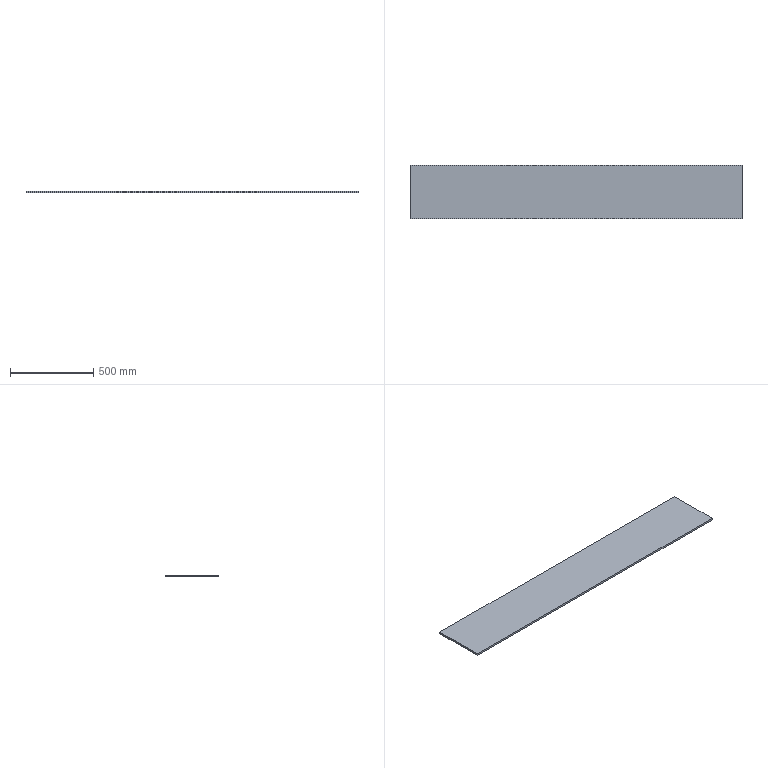Component | SolidWorks | TopCover-1 | 1 solid | 6 faces | box 2000 x 320 x 12 mm | volume 7680000 mm3 | plane 6 | material Plain Carbon Steel
STEP:
#1=COLOUR_RGB('',0.7922,0.8196,0.9333);
#2=FILL_AREA_STYLE_COLOUR('',#1);
#3=FILL_AREA_STYLE('',(#2));
#4=SURFACE_STYLE_FILL_AREA(#3);
#5=SURFACE_SIDE_STYLE('',(#4));
#6=SURFACE_STYLE_USAGE(.BOTH.,#5);
#7=PRESENTATION_STYLE_ASSIGNMENT((#6));
#8=CARTESIAN_POINT('',(88.605,43.163,65.555));
#9=VERTEX_POINT('',#8);
#10=CARTESIAN_POINT('',(88.605,55.762,65.555));
#11=VERTEX_POINT('',#10);
#12=CARTESIAN_POINT('',(88.605,55.762,65.555));
#13=DIRECTION('',(0.,1.,0.));
#14=VECTOR('',#13,39.37);
#15=LINE('',#12,#14);
#16=EDGE_CURVE('',#9,#11,#15,.T.);
#17=ORIENTED_EDGE('',*,*,#16,.F.);
#18=CARTESIAN_POINT('',(88.605,43.163,65.082));
#19=VERTEX_POINT('',#18);
#20=CARTESIAN_POINT('',(88.605,43.163,65.082));
#21=DIRECTION('',(0.,-0.,1.));
#22=VECTOR('',#21,39.37);
#23=LINE('',#20,#22);
#24=EDGE_CURVE('',#19,#9,#23,.T.);
#25=ORIENTED_EDGE('',*,*,#24,.F.);
#26=CARTESIAN_POINT('',(88.605,55.762,65.082));
#27=VERTEX_POINT('',#26);
#28=CARTESIAN_POINT('',(88.605,55.762,65.082));
#29=DIRECTION('',(0.,1.,0.));
#30=VECTOR('',#29,39.37);
#31=LINE('',#28,#30);
#32=EDGE_CURVE('',#19,#27,#31,.T.);
#33=ORIENTED_EDGE('',*,*,#32,.T.);
#34=CARTESIAN_POINT('',(88.605,55.762,65.082));
#35=DIRECTION('',(0.,-0.,1.));
#36=VECTOR('',#35,39.37);
#37=LINE('',#34,#36);
#38=EDGE_CURVE('',#27,#11,#37,.T.);
#39=ORIENTED_EDGE('',*,*,#38,.T.);
#40=EDGE_LOOP('',(#17,#25,#33,#39));
#41=FACE_OUTER_BOUND('',#40,.T.);
#42=CARTESIAN_POINT('',(88.605,55.762,65.082));
#43=DIRECTION('',(1.,0.,0.));
#44=DIRECTION('',(0.,1.,0.));
#45=AXIS2_PLACEMENT_3D('',#42,#43,#44);
#46=PLANE('',#45);
#47=ADVANCED_FACE('',(#41),#46,.T.);
#48=CARTESIAN_POINT('',(9.865,43.163,65.555));
#49=VERTEX_POINT('',#48);
#50=CARTESIAN_POINT('',(9.865,43.163,65.555));
#51=DIRECTION('',(1.,0.,0.));
#52=VECTOR('',#51,39.37);
#53=LINE('',#50,#52);
#54=EDGE_CURVE('',#49,#9,#53,.T.);
#55=ORIENTED_EDGE('',*,*,#54,.F.);
#56=CARTESIAN_POINT('',(9.865,43.163,65.082));
#57=VERTEX_POINT('',#56);
#58=CARTESIAN_POINT('',(9.865,43.163,65.082));
#59=DIRECTION('',(0.,-0.,1.));
#60=VECTOR('',#59,39.37);
#61=LINE('',#58,#60);
#62=EDGE_CURVE('',#57,#49,#61,.T.);
#63=ORIENTED_EDGE('',*,*,#62,.F.);
#64=CARTESIAN_POINT('',(9.865,43.163,65.082));
#65=DIRECTION('',(1.,0.,0.));
#66=VECTOR('',#65,39.37);
#67=LINE('',#64,#66);
#68=EDGE_CURVE('',#57,#19,#67,.T.);
#69=ORIENTED_EDGE('',*,*,#68,.T.);
#70=ORIENTED_EDGE('',*,*,#24,.T.);
#71=EDGE_LOOP('',(#55,#63,#69,#70));
#72=FACE_OUTER_BOUND('',#71,.T.);
#73=CARTESIAN_POINT('',(9.865,43.163,65.082));
#74=DIRECTION('',(0.,-1.,-0.));
#75=DIRECTION('',(1.,0.,0.));
#76=AXIS2_PLACEMENT_3D('',#73,#74,#75);
#77=PLANE('',#76);
#78=ADVANCED_FACE('',(#72),#77,.T.);
#79=CARTESIAN_POINT('',(9.865,55.762,65.555));
#80=VERTEX_POINT('',#79);
#81=CARTESIAN_POINT('',(9.865,55.762,65.555));
#82=DIRECTION('',(0.,-1.,-0.));
#83=VECTOR('',#82,39.37);
#84=LINE('',#81,#83);
#85=EDGE_CURVE('',#80,#49,#84,.T.);
#86=ORIENTED_EDGE('',*,*,#85,.F.);
#87=CARTESIAN_POINT('',(9.865,55.762,65.082));
#88=VERTEX_POINT('',#87);
#89=CARTESIAN_POINT('',(9.865,55.762,65.082));
#90=DIRECTION('',(0.,-0.,1.));
#91=VECTOR('',#90,39.37);
#92=LINE('',#89,#91);
#93=EDGE_CURVE('',#88,#80,#92,.T.);
#94=ORIENTED_EDGE('',*,*,#93,.F.);
#95=CARTESIAN_POINT('',(9.865,55.762,65.082));
#96=DIRECTION('',(0.,-1.,-0.));
#97=VECTOR('',#96,39.37);
#98=LINE('',#95,#97);
#99=EDGE_CURVE('',#88,#57,#98,.T.);
#100=ORIENTED_EDGE('',*,*,#99,.T.);
#101=ORIENTED_EDGE('',*,*,#62,.T.);
#102=EDGE_LOOP('',(#86,#94,#100,#101));
#103=FACE_OUTER_BOUND('',#102,.T.);
#104=CARTESIAN_POINT('',(9.865,55.762,65.082));
#105=DIRECTION('',(-1.,0.,0.));
#106=DIRECTION('',(0.,-1.,-0.));
#107=AXIS2_PLACEMENT_3D('',#104,#105,#106);
#108=PLANE('',#107);
#109=ADVANCED_FACE('',(#103),#108,.T.);
#110=CARTESIAN_POINT('',(9.865,55.762,65.555));
#111=DIRECTION('',(-1.,0.,0.));
#112=VECTOR('',#111,39.37);
#113=LINE('',#110,#112);
#114=EDGE_CURVE('',#11,#80,#113,.T.);
#115=ORIENTED_EDGE('',*,*,#114,.F.);
#116=ORIENTED_EDGE('',*,*,#38,.F.);
#117=CARTESIAN_POINT('',(9.865,55.762,65.082));
#118=DIRECTION('',(-1.,0.,0.));
#119=VECTOR('',#118,39.37);
#120=LINE('',#117,#119);
#121=EDGE_CURVE('',#27,#88,#120,.T.);
#122=ORIENTED_EDGE('',*,*,#121,.T.);
#123=ORIENTED_EDGE('',*,*,#93,.T.);
#124=EDGE_LOOP('',(#115,#116,#122,#123));
#125=FACE_OUTER_BOUND('',#124,.T.);
#126=CARTESIAN_POINT('',(9.865,55.762,65.082));
#127=DIRECTION('',(0.,1.,0.));
#128=DIRECTION('',(-1.,0.,0.));
#129=AXIS2_PLACEMENT_3D('',#126,#127,#128);
#130=PLANE('',#129);
#131=ADVANCED_FACE('',(#125),#130,.T.);
#132=ORIENTED_EDGE('',*,*,#32,.F.);
#133=ORIENTED_EDGE('',*,*,#68,.F.);
#134=ORIENTED_EDGE('',*,*,#99,.F.);
#135=ORIENTED_EDGE('',*,*,#121,.F.);
#136=EDGE_LOOP('',(#132,#133,#134,#135));
#137=FACE_OUTER_BOUND('',#136,.T.);
#138=CARTESIAN_POINT('',(49.235,49.463,65.082));
#139=DIRECTION('',(0.,-0.,1.));
#140=DIRECTION('',(0.,-1.,-0.));
#141=AXIS2_PLACEMENT_3D('',#138,#139,#140);
#142=PLANE('',#141);
#143=ADVANCED_FACE('',(#137),#142,.F.);
#144=ORIENTED_EDGE('',*,*,#16,.T.);
#145=ORIENTED_EDGE('',*,*,#114,.T.);
#146=ORIENTED_EDGE('',*,*,#85,.T.);
#147=ORIENTED_EDGE('',*,*,#54,.T.);
#148=EDGE_LOOP('',(#144,#145,#146,#147));
#149=FACE_OUTER_BOUND('',#148,.T.);
#150=CARTESIAN_POINT('',(49.235,49.463,65.555));
#151=DIRECTION('',(0.,-0.,1.));
#152=DIRECTION('',(0.,-1.,-0.));
#153=AXIS2_PLACEMENT_3D('',#150,#151,#152);
#154=PLANE('',#153);
#155=ADVANCED_FACE('',(#149),#154,.T.);
#156=CLOSED_SHELL('',(#47,#78,#109,#131,#143,#155));
#157=MANIFOLD_SOLID_BREP('',#156);
#158=STYLED_ITEM('',(#7),#157);
#159=(LENGTH_UNIT()NAMED_UNIT(*)SI_UNIT($,.METRE.));
#160=LENGTH_MEASURE_WITH_UNIT(LENGTH_MEASURE(0.0254),#159);
#161=DIMENSIONAL_EXPONENTS(1.,0.,0.,0.,0.,0.,0.);
#162=(CONVERSION_BASED_UNIT('',#160)LENGTH_UNIT()NAMED_UNIT(#161));
#163=UNCERTAINTY_MEASURE_WITH_UNIT(LENGTH_MEASURE(0.00001),#162,'','');
#164=(NAMED_UNIT(*)PLANE_ANGLE_UNIT()SI_UNIT($,.RADIAN.));
#165=(NAMED_UNIT(*)SI_UNIT($,.STERADIAN.)SOLID_ANGLE_UNIT());
#166=(GEOMETRIC_REPRESENTATION_CONTEXT(3)GLOBAL_UNCERTAINTY_ASSIGNED_CONTEXT((#163))GLOBAL_UNIT_ASSIGNED_CONTEXT((#162,#164,#165))REPRESENTATION_CONTEXT('',''));
#167=MECHANICAL_DESIGN_GEOMETRIC_PRESENTATION_REPRESENTATION('',(#158),#166);
#168=PRESENTATION_LAYER_ASSIGNMENT('','',(#158));
#169=CARTESIAN_POINT('',(0.,0.,0.));
#170=DIRECTION('',(0.,0.,1.));
#171=DIRECTION('',(1.,0.,0.));
#172=AXIS2_PLACEMENT_3D('',#169,#170,#171);
#173=(LENGTH_UNIT()NAMED_UNIT(*)SI_UNIT($,.METRE.));
#174=LENGTH_MEASURE_WITH_UNIT(LENGTH_MEASURE(0.0254),#173);
#175=DIMENSIONAL_EXPONENTS(1.,0.,0.,0.,0.,0.,0.);
#176=(CONVERSION_BASED_UNIT('',#174)LENGTH_UNIT()NAMED_UNIT(#175));
#177=UNCERTAINTY_MEASURE_WITH_UNIT(LENGTH_MEASURE(0.00001),#176,'','');
#178=(NAMED_UNIT(*)PLANE_ANGLE_UNIT()SI_UNIT($,.RADIAN.));
#179=(NAMED_UNIT(*)SI_UNIT($,.STERADIAN.)SOLID_ANGLE_UNIT());
#180=(GEOMETRIC_REPRESENTATION_CONTEXT(3)GLOBAL_UNCERTAINTY_ASSIGNED_CONTEXT((#177))GLOBAL_UNIT_ASSIGNED_CONTEXT((#176,#178,#179))REPRESENTATION_CONTEXT('',''));
#181=ADVANCED_BREP_SHAPE_REPRESENTATION('',(#157,#172),#180);